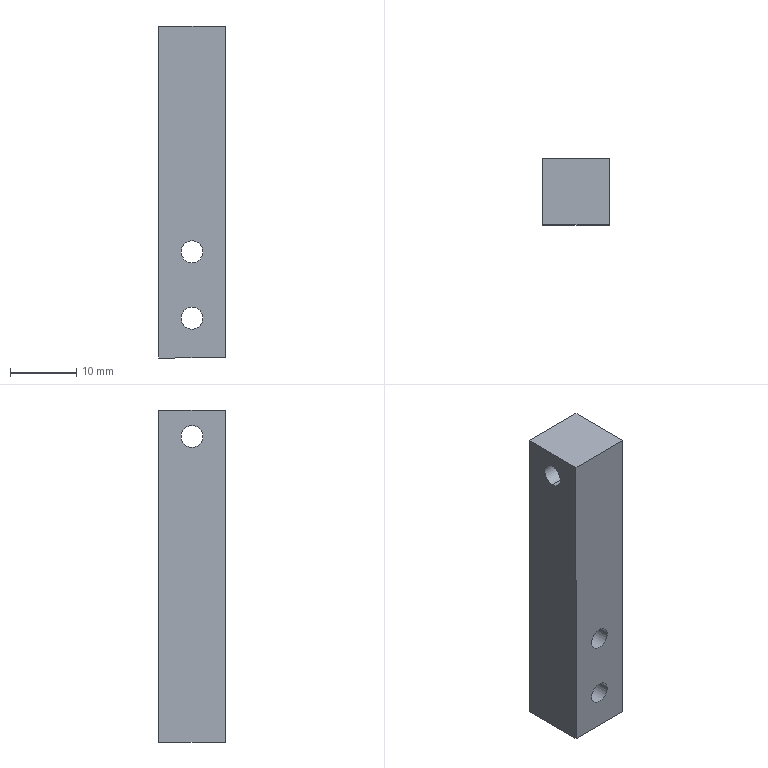Component | SolidWorks | CS021-A10-A024-1 | 1 solid | 12 faces | box 10 x 10 x 50 mm | volume 4743 mm3 | cylinder 6 | plane 6 | commonest cylinder face diameters 3.3 x6 | material AL6061
build123d program:
from build123d import *

# Parameters (mm, degrees)
SKETCH1_W                  = 50
SKETCH1_H                  = 10
BOSS_EXTRUDE1_DEPTH        = 5
F_3_3_3_3_DIAMETER_HOLE1_D = 3.3
M4_TAPPED_HOLE1_D          = 3.3


with BuildPart() as part:
    # Sketch1 → Boss-Extrude1 (new, symmetric)
    with BuildSketch(Plane.XY):
        Rectangle(SKETCH1_W, SKETCH1_H)
    extrude(amount=BOSS_EXTRUDE1_DEPTH, both=True)

    # 3.3 _3.3_ Diameter Hole1 (through all)
    with Locations(Plane(origin=(0, 5, 0), x_dir=(1, 0, 0), z_dir=(0, 1, 0))):
        with Locations((19, 0), (9, 0)):
            Hole(F_3_3_3_3_DIAMETER_HOLE1_D / 2)

    # M4 Tapped Hole1 (through all)
    with Locations(Plane.XY.offset(5)):
        with Locations((-21, 0)):
            Hole(M4_TAPPED_HOLE1_D / 2)


solid = part.part

# Placed as in the assembly
solid = solid.moved(Location((172.449, 93.817, -71), (0, 90, 0)))
STEP:
#1=CARTESIAN_POINT('',(6.592,3.694,-1.904));
#2=VERTEX_POINT('',#1);
#3=CARTESIAN_POINT('',(6.592,3.694,-2.033));
#4=VERTEX_POINT('',#3);
#5=CARTESIAN_POINT('',(6.592,3.694,-1.969));
#6=DIRECTION('',(1.,-0.,0.));
#7=DIRECTION('',(0.,0.,-1.));
#8=AXIS2_PLACEMENT_3D('',#5,#6,#7);
#9=CIRCLE('',#8,0.06496);
#10=EDGE_CURVE('',#2,#4,#9,.T.);
#11=ORIENTED_EDGE('',*,*,#10,.F.);
#12=CARTESIAN_POINT('',(6.986,3.694,-1.904));
#13=VERTEX_POINT('',#12);
#14=CARTESIAN_POINT('',(6.986,3.694,-1.904));
#15=DIRECTION('',(1.,-0.,0.));
#16=VECTOR('',#15,39.37);
#17=LINE('',#14,#16);
#18=EDGE_CURVE('',#2,#13,#17,.T.);
#19=ORIENTED_EDGE('',*,*,#18,.T.);
#20=CARTESIAN_POINT('',(6.986,3.694,-2.033));
#21=VERTEX_POINT('',#20);
#22=CARTESIAN_POINT('',(6.986,3.694,-1.969));
#23=DIRECTION('',(1.,-0.,0.));
#24=DIRECTION('',(0.,0.,-1.));
#25=AXIS2_PLACEMENT_3D('',#22,#23,#24);
#26=CIRCLE('',#25,0.06496);
#27=EDGE_CURVE('',#13,#21,#26,.T.);
#28=ORIENTED_EDGE('',*,*,#27,.T.);
#29=CARTESIAN_POINT('',(6.986,3.694,-2.033));
#30=DIRECTION('',(1.,-0.,0.));
#31=VECTOR('',#30,39.37);
#32=LINE('',#29,#31);
#33=EDGE_CURVE('',#4,#21,#32,.T.);
#34=ORIENTED_EDGE('',*,*,#33,.F.);
#35=EDGE_LOOP('',(#11,#19,#28,#34));
#36=FACE_OUTER_BOUND('',#35,.T.);
#37=CARTESIAN_POINT('',(6.986,3.694,-1.969));
#38=DIRECTION('',(1.,-0.,0.));
#39=DIRECTION('',(0.,0.,-1.));
#40=AXIS2_PLACEMENT_3D('',#37,#38,#39);
#41=CYLINDRICAL_SURFACE('',#40,0.06496);
#42=ADVANCED_FACE('',(#36),#41,.F.);
#43=CARTESIAN_POINT('',(6.724,3.497,-3.543));
#44=VERTEX_POINT('',#43);
#45=CARTESIAN_POINT('',(6.854,3.497,-3.543));
#46=VERTEX_POINT('',#45);
#47=CARTESIAN_POINT('',(6.789,3.497,-3.543));
#48=DIRECTION('',(0.,1.,-0.));
#49=DIRECTION('',(1.,0.,0.));
#50=AXIS2_PLACEMENT_3D('',#47,#48,#49);
#51=CIRCLE('',#50,0.06496);
#52=EDGE_CURVE('',#44,#46,#51,.T.);
#53=ORIENTED_EDGE('',*,*,#52,.F.);
#54=CARTESIAN_POINT('',(6.724,3.89,-3.543));
#55=VERTEX_POINT('',#54);
#56=CARTESIAN_POINT('',(6.724,3.89,-3.543));
#57=DIRECTION('',(0.,1.,-0.));
#58=VECTOR('',#57,39.37);
#59=LINE('',#56,#58);
#60=EDGE_CURVE('',#44,#55,#59,.T.);
#61=ORIENTED_EDGE('',*,*,#60,.T.);
#62=CARTESIAN_POINT('',(6.854,3.89,-3.543));
#63=VERTEX_POINT('',#62);
#64=CARTESIAN_POINT('',(6.789,3.89,-3.543));
#65=DIRECTION('',(0.,1.,-0.));
#66=DIRECTION('',(1.,0.,0.));
#67=AXIS2_PLACEMENT_3D('',#64,#65,#66);
#68=CIRCLE('',#67,0.06496);
#69=EDGE_CURVE('',#55,#63,#68,.T.);
#70=ORIENTED_EDGE('',*,*,#69,.T.);
#71=CARTESIAN_POINT('',(6.854,3.89,-3.543));
#72=DIRECTION('',(0.,1.,-0.));
#73=VECTOR('',#72,39.37);
#74=LINE('',#71,#73);
#75=EDGE_CURVE('',#46,#63,#74,.T.);
#76=ORIENTED_EDGE('',*,*,#75,.F.);
#77=EDGE_LOOP('',(#53,#61,#70,#76));
#78=FACE_OUTER_BOUND('',#77,.T.);
#79=CARTESIAN_POINT('',(6.789,3.89,-3.543));
#80=DIRECTION('',(0.,1.,-0.));
#81=DIRECTION('',(1.,0.,0.));
#82=AXIS2_PLACEMENT_3D('',#79,#80,#81);
#83=CYLINDRICAL_SURFACE('',#82,0.06496);
#84=ADVANCED_FACE('',(#78),#83,.F.);
#85=CARTESIAN_POINT('',(6.724,3.497,-3.15));
#86=VERTEX_POINT('',#85);
#87=CARTESIAN_POINT('',(6.854,3.497,-3.15));
#88=VERTEX_POINT('',#87);
#89=CARTESIAN_POINT('',(6.789,3.497,-3.15));
#90=DIRECTION('',(0.,1.,-0.));
#91=DIRECTION('',(1.,0.,0.));
#92=AXIS2_PLACEMENT_3D('',#89,#90,#91);
#93=CIRCLE('',#92,0.06496);
#94=EDGE_CURVE('',#86,#88,#93,.T.);
#95=ORIENTED_EDGE('',*,*,#94,.F.);
#96=CARTESIAN_POINT('',(6.724,3.89,-3.15));
#97=VERTEX_POINT('',#96);
#98=CARTESIAN_POINT('',(6.724,3.89,-3.15));
#99=DIRECTION('',(0.,1.,-0.));
#100=VECTOR('',#99,39.37);
#101=LINE('',#98,#100);
#102=EDGE_CURVE('',#86,#97,#101,.T.);
#103=ORIENTED_EDGE('',*,*,#102,.T.);
#104=CARTESIAN_POINT('',(6.854,3.89,-3.15));
#105=VERTEX_POINT('',#104);
#106=CARTESIAN_POINT('',(6.789,3.89,-3.15));
#107=DIRECTION('',(0.,1.,-0.));
#108=DIRECTION('',(1.,0.,0.));
#109=AXIS2_PLACEMENT_3D('',#106,#107,#108);
#110=CIRCLE('',#109,0.06496);
#111=EDGE_CURVE('',#97,#105,#110,.T.);
#112=ORIENTED_EDGE('',*,*,#111,.T.);
#113=CARTESIAN_POINT('',(6.854,3.89,-3.15));
#114=DIRECTION('',(0.,1.,-0.));
#115=VECTOR('',#114,39.37);
#116=LINE('',#113,#115);
#117=EDGE_CURVE('',#88,#105,#116,.T.);
#118=ORIENTED_EDGE('',*,*,#117,.F.);
#119=EDGE_LOOP('',(#95,#103,#112,#118));
#120=FACE_OUTER_BOUND('',#119,.T.);
#121=CARTESIAN_POINT('',(6.789,3.89,-3.15));
#122=DIRECTION('',(0.,1.,-0.));
#123=DIRECTION('',(1.,0.,0.));
#124=AXIS2_PLACEMENT_3D('',#121,#122,#123);
#125=CYLINDRICAL_SURFACE('',#124,0.06496);
#126=ADVANCED_FACE('',(#120),#125,.F.);
#127=CARTESIAN_POINT('',(6.592,3.497,-3.78));
#128=VERTEX_POINT('',#127);
#129=CARTESIAN_POINT('',(6.592,3.89,-3.78));
#130=VERTEX_POINT('',#129);
#131=CARTESIAN_POINT('',(6.592,3.497,-3.78));
#132=DIRECTION('',(0.,1.,-0.));
#133=VECTOR('',#132,39.37);
#134=LINE('',#131,#133);
#135=EDGE_CURVE('',#128,#130,#134,.T.);
#136=ORIENTED_EDGE('',*,*,#135,.T.);
#137=CARTESIAN_POINT('',(6.986,3.89,-3.78));
#138=VERTEX_POINT('',#137);
#139=CARTESIAN_POINT('',(6.986,3.89,-3.78));
#140=DIRECTION('',(-1.,0.,-0.));
#141=VECTOR('',#140,39.37);
#142=LINE('',#139,#141);
#143=EDGE_CURVE('',#138,#130,#142,.T.);
#144=ORIENTED_EDGE('',*,*,#143,.F.);
#145=CARTESIAN_POINT('',(6.986,3.497,-3.78));
#146=VERTEX_POINT('',#145);
#147=CARTESIAN_POINT('',(6.986,3.497,-3.78));
#148=DIRECTION('',(0.,1.,-0.));
#149=VECTOR('',#148,39.37);
#150=LINE('',#147,#149);
#151=EDGE_CURVE('',#146,#138,#150,.T.);
#152=ORIENTED_EDGE('',*,*,#151,.F.);
#153=CARTESIAN_POINT('',(6.986,3.497,-3.78));
#154=DIRECTION('',(-1.,0.,-0.));
#155=VECTOR('',#154,39.37);
#156=LINE('',#153,#155);
#157=EDGE_CURVE('',#146,#128,#156,.T.);
#158=ORIENTED_EDGE('',*,*,#157,.T.);
#159=EDGE_LOOP('',(#136,#144,#152,#158));
#160=FACE_OUTER_BOUND('',#159,.T.);
#161=CARTESIAN_POINT('',(6.986,3.497,-3.78));
#162=DIRECTION('',(-0.,0.,1.));
#163=DIRECTION('',(1.,-0.,0.));
#164=AXIS2_PLACEMENT_3D('',#161,#162,#163);
#165=PLANE('',#164);
#166=ADVANCED_FACE('',(#160),#165,.F.);
#167=CARTESIAN_POINT('',(6.789,3.89,-3.543));
#168=DIRECTION('',(0.,1.,-0.));
#169=DIRECTION('',(1.,0.,0.));
#170=AXIS2_PLACEMENT_3D('',#167,#168,#169);
#171=CIRCLE('',#170,0.06496);
#172=EDGE_CURVE('',#63,#55,#171,.T.);
#173=ORIENTED_EDGE('',*,*,#172,.F.);
#174=ORIENTED_EDGE('',*,*,#69,.F.);
#175=EDGE_LOOP('',(#173,#174));
#176=FACE_BOUND('',#175,.T.);
#177=CARTESIAN_POINT('',(6.789,3.89,-3.15));
#178=DIRECTION('',(0.,1.,-0.));
#179=DIRECTION('',(1.,0.,0.));
#180=AXIS2_PLACEMENT_3D('',#177,#178,#179);
#181=CIRCLE('',#180,0.06496);
#182=EDGE_CURVE('',#105,#97,#181,.T.);
#183=ORIENTED_EDGE('',*,*,#182,.F.);
#184=ORIENTED_EDGE('',*,*,#111,.F.);
#185=EDGE_LOOP('',(#183,#184));
#186=FACE_BOUND('',#185,.T.);
#187=CARTESIAN_POINT('',(6.592,3.89,-1.811));
#188=VERTEX_POINT('',#187);
#189=CARTESIAN_POINT('',(6.592,3.89,-1.811));
#190=DIRECTION('',(-0.,0.,1.));
#191=VECTOR('',#190,39.37);
#192=LINE('',#189,#191);
#193=EDGE_CURVE('',#130,#188,#192,.T.);
#194=ORIENTED_EDGE('',*,*,#193,.T.);
#195=CARTESIAN_POINT('',(6.986,3.89,-1.811));
#196=VERTEX_POINT('',#195);
#197=CARTESIAN_POINT('',(6.986,3.89,-1.811));
#198=DIRECTION('',(-1.,0.,-0.));
#199=VECTOR('',#198,39.37);
#200=LINE('',#197,#199);
#201=EDGE_CURVE('',#196,#188,#200,.T.);
#202=ORIENTED_EDGE('',*,*,#201,.F.);
#203=CARTESIAN_POINT('',(6.986,3.89,-1.811));
#204=DIRECTION('',(-0.,0.,1.));
#205=VECTOR('',#204,39.37);
#206=LINE('',#203,#205);
#207=EDGE_CURVE('',#138,#196,#206,.T.);
#208=ORIENTED_EDGE('',*,*,#207,.F.);
#209=ORIENTED_EDGE('',*,*,#143,.T.);
#210=EDGE_LOOP('',(#194,#202,#208,#209));
#211=FACE_OUTER_BOUND('',#210,.T.);
#212=CARTESIAN_POINT('',(6.986,3.89,-1.811));
#213=DIRECTION('',(-0.,-1.,0.));
#214=DIRECTION('',(-1.,0.,-0.));
#215=AXIS2_PLACEMENT_3D('',#212,#213,#214);
#216=PLANE('',#215);
#217=ADVANCED_FACE('',(#176,#186,#211),#216,.F.);
#218=CARTESIAN_POINT('',(6.592,3.497,-1.811));
#219=VERTEX_POINT('',#218);
#220=CARTESIAN_POINT('',(6.592,3.497,-1.811));
#221=DIRECTION('',(-0.,-1.,0.));
#222=VECTOR('',#221,39.37);
#223=LINE('',#220,#222);
#224=EDGE_CURVE('',#188,#219,#223,.T.);
#225=ORIENTED_EDGE('',*,*,#224,.T.);
#226=CARTESIAN_POINT('',(6.986,3.497,-1.811));
#227=VERTEX_POINT('',#226);
#228=CARTESIAN_POINT('',(6.986,3.497,-1.811));
#229=DIRECTION('',(-1.,0.,-0.));
#230=VECTOR('',#229,39.37);
#231=LINE('',#228,#230);
#232=EDGE_CURVE('',#227,#219,#231,.T.);
#233=ORIENTED_EDGE('',*,*,#232,.F.);
#234=CARTESIAN_POINT('',(6.986,3.497,-1.811));
#235=DIRECTION('',(-0.,-1.,0.));
#236=VECTOR('',#235,39.37);
#237=LINE('',#234,#236);
#238=EDGE_CURVE('',#196,#227,#237,.T.);
#239=ORIENTED_EDGE('',*,*,#238,.F.);
#240=ORIENTED_EDGE('',*,*,#201,.T.);
#241=EDGE_LOOP('',(#225,#233,#239,#240));
#242=FACE_OUTER_BOUND('',#241,.T.);
#243=CARTESIAN_POINT('',(6.986,3.497,-1.811));
#244=DIRECTION('',(0.,-0.,-1.));
#245=DIRECTION('',(-1.,0.,-0.));
#246=AXIS2_PLACEMENT_3D('',#243,#244,#245);
#247=PLANE('',#246);
#248=ADVANCED_FACE('',(#242),#247,.F.);
#249=CARTESIAN_POINT('',(6.789,3.497,-3.543));
#250=DIRECTION('',(0.,1.,-0.));
#251=DIRECTION('',(1.,0.,0.));
#252=AXIS2_PLACEMENT_3D('',#249,#250,#251);
#253=CIRCLE('',#252,0.06496);
#254=EDGE_CURVE('',#46,#44,#253,.T.);
#255=ORIENTED_EDGE('',*,*,#254,.T.);
#256=ORIENTED_EDGE('',*,*,#52,.T.);
#257=EDGE_LOOP('',(#255,#256));
#258=FACE_BOUND('',#257,.T.);
#259=CARTESIAN_POINT('',(6.789,3.497,-3.15));
#260=DIRECTION('',(0.,1.,-0.));
#261=DIRECTION('',(1.,0.,0.));
#262=AXIS2_PLACEMENT_3D('',#259,#260,#261);
#263=CIRCLE('',#262,0.06496);
#264=EDGE_CURVE('',#88,#86,#263,.T.);
#265=ORIENTED_EDGE('',*,*,#264,.T.);
#266=ORIENTED_EDGE('',*,*,#94,.T.);
#267=EDGE_LOOP('',(#265,#266));
#268=FACE_BOUND('',#267,.T.);
#269=CARTESIAN_POINT('',(6.592,3.497,-1.811));
#270=DIRECTION('',(0.,-0.,-1.));
#271=VECTOR('',#270,39.37);
#272=LINE('',#269,#271);
#273=EDGE_CURVE('',#219,#128,#272,.T.);
#274=ORIENTED_EDGE('',*,*,#273,.T.);
#275=ORIENTED_EDGE('',*,*,#157,.F.);
#276=CARTESIAN_POINT('',(6.986,3.497,-1.811));
#277=DIRECTION('',(0.,-0.,-1.));
#278=VECTOR('',#277,39.37);
#279=LINE('',#276,#278);
#280=EDGE_CURVE('',#227,#146,#279,.T.);
#281=ORIENTED_EDGE('',*,*,#280,.F.);
#282=ORIENTED_EDGE('',*,*,#232,.T.);
#283=EDGE_LOOP('',(#274,#275,#281,#282));
#284=FACE_OUTER_BOUND('',#283,.T.);
#285=CARTESIAN_POINT('',(6.986,3.497,-1.811));
#286=DIRECTION('',(0.,1.,-0.));
#287=DIRECTION('',(1.,-0.,0.));
#288=AXIS2_PLACEMENT_3D('',#285,#286,#287);
#289=PLANE('',#288);
#290=ADVANCED_FACE('',(#258,#268,#284),#289,.F.);
#291=CARTESIAN_POINT('',(6.986,3.694,-1.969));
#292=DIRECTION('',(1.,-0.,0.));
#293=DIRECTION('',(0.,0.,-1.));
#294=AXIS2_PLACEMENT_3D('',#291,#292,#293);
#295=CIRCLE('',#294,0.06496);
#296=EDGE_CURVE('',#21,#13,#295,.T.);
#297=ORIENTED_EDGE('',*,*,#296,.F.);
#298=ORIENTED_EDGE('',*,*,#27,.F.);
#299=EDGE_LOOP('',(#297,#298));
#300=FACE_BOUND('',#299,.T.);
#301=ORIENTED_EDGE('',*,*,#151,.T.);
#302=ORIENTED_EDGE('',*,*,#207,.T.);
#303=ORIENTED_EDGE('',*,*,#238,.T.);
#304=ORIENTED_EDGE('',*,*,#280,.T.);
#305=EDGE_LOOP('',(#301,#302,#303,#304));
#306=FACE_OUTER_BOUND('',#305,.T.);
#307=CARTESIAN_POINT('',(6.986,3.694,-2.795));
#308=DIRECTION('',(-1.,0.,-0.));
#309=DIRECTION('',(-0.,0.,1.));
#310=AXIS2_PLACEMENT_3D('',#307,#308,#309);
#311=PLANE('',#310);
#312=ADVANCED_FACE('',(#300,#306),#311,.F.);
#313=CARTESIAN_POINT('',(6.592,3.694,-1.969));
#314=DIRECTION('',(1.,-0.,0.));
#315=DIRECTION('',(0.,0.,-1.));
#316=AXIS2_PLACEMENT_3D('',#313,#314,#315);
#317=CIRCLE('',#316,0.06496);
#318=EDGE_CURVE('',#4,#2,#317,.T.);
#319=ORIENTED_EDGE('',*,*,#318,.T.);
#320=ORIENTED_EDGE('',*,*,#10,.T.);
#321=EDGE_LOOP('',(#319,#320));
#322=FACE_BOUND('',#321,.T.);
#323=ORIENTED_EDGE('',*,*,#135,.F.);
#324=ORIENTED_EDGE('',*,*,#273,.F.);
#325=ORIENTED_EDGE('',*,*,#224,.F.);
#326=ORIENTED_EDGE('',*,*,#193,.F.);
#327=EDGE_LOOP('',(#323,#324,#325,#326));
#328=FACE_OUTER_BOUND('',#327,.T.);
#329=CARTESIAN_POINT('',(6.592,3.694,-2.795));
#330=DIRECTION('',(-1.,0.,-0.));
#331=DIRECTION('',(-0.,0.,1.));
#332=AXIS2_PLACEMENT_3D('',#329,#330,#331);
#333=PLANE('',#332);
#334=ADVANCED_FACE('',(#322,#328),#333,.T.);
#335=ORIENTED_EDGE('',*,*,#102,.F.);
#336=ORIENTED_EDGE('',*,*,#264,.F.);
#337=ORIENTED_EDGE('',*,*,#117,.T.);
#338=ORIENTED_EDGE('',*,*,#182,.T.);
#339=EDGE_LOOP('',(#335,#336,#337,#338));
#340=FACE_OUTER_BOUND('',#339,.T.);
#341=CARTESIAN_POINT('',(6.789,3.89,-3.15));
#342=DIRECTION('',(0.,1.,-0.));
#343=DIRECTION('',(1.,0.,0.));
#344=AXIS2_PLACEMENT_3D('',#341,#342,#343);
#345=CYLINDRICAL_SURFACE('',#344,0.06496);
#346=ADVANCED_FACE('',(#340),#345,.F.);
#347=ORIENTED_EDGE('',*,*,#60,.F.);
#348=ORIENTED_EDGE('',*,*,#254,.F.);
#349=ORIENTED_EDGE('',*,*,#75,.T.);
#350=ORIENTED_EDGE('',*,*,#172,.T.);
#351=EDGE_LOOP('',(#347,#348,#349,#350));
#352=FACE_OUTER_BOUND('',#351,.T.);
#353=CARTESIAN_POINT('',(6.789,3.89,-3.543));
#354=DIRECTION('',(0.,1.,-0.));
#355=DIRECTION('',(1.,0.,0.));
#356=AXIS2_PLACEMENT_3D('',#353,#354,#355);
#357=CYLINDRICAL_SURFACE('',#356,0.06496);
#358=ADVANCED_FACE('',(#352),#357,.F.);
#359=ORIENTED_EDGE('',*,*,#18,.F.);
#360=ORIENTED_EDGE('',*,*,#318,.F.);
#361=ORIENTED_EDGE('',*,*,#33,.T.);
#362=ORIENTED_EDGE('',*,*,#296,.T.);
#363=EDGE_LOOP('',(#359,#360,#361,#362));
#364=FACE_OUTER_BOUND('',#363,.T.);
#365=CARTESIAN_POINT('',(6.986,3.694,-1.969));
#366=DIRECTION('',(1.,-0.,0.));
#367=DIRECTION('',(0.,0.,-1.));
#368=AXIS2_PLACEMENT_3D('',#365,#366,#367);
#369=CYLINDRICAL_SURFACE('',#368,0.06496);
#370=ADVANCED_FACE('',(#364),#369,.F.);
#371=CLOSED_SHELL('',(#42,#84,#126,#166,#217,#248,#290,#312,#334,#346,#358,#370));
#372=MANIFOLD_SOLID_BREP('',#371);
#373=CARTESIAN_POINT('',(0.,0.,0.));
#374=DIRECTION('',(0.,0.,1.));
#375=DIRECTION('',(1.,0.,0.));
#376=AXIS2_PLACEMENT_3D('',#373,#374,#375);
#377=(LENGTH_UNIT()NAMED_UNIT(*)SI_UNIT($,.METRE.));
#378=LENGTH_MEASURE_WITH_UNIT(LENGTH_MEASURE(0.0254),#377);
#379=DIMENSIONAL_EXPONENTS(1.,0.,0.,0.,0.,0.,0.);
#380=(CONVERSION_BASED_UNIT('',#378)LENGTH_UNIT()NAMED_UNIT(#379));
#381=UNCERTAINTY_MEASURE_WITH_UNIT(LENGTH_MEASURE(0.00001),#380,'','');
#382=(NAMED_UNIT(*)PLANE_ANGLE_UNIT()SI_UNIT($,.RADIAN.));
#383=(NAMED_UNIT(*)SI_UNIT($,.STERADIAN.)SOLID_ANGLE_UNIT());
#384=(GEOMETRIC_REPRESENTATION_CONTEXT(3)GLOBAL_UNCERTAINTY_ASSIGNED_CONTEXT((#381))GLOBAL_UNIT_ASSIGNED_CONTEXT((#380,#382,#383))REPRESENTATION_CONTEXT('',''));
#385=ADVANCED_BREP_SHAPE_REPRESENTATION('',(#372,#376),#384);
#386=COLOUR_RGB('',0.7922,0.8196,0.9333);
#387=FILL_AREA_STYLE_COLOUR('',#386);
#388=FILL_AREA_STYLE('',(#387));
#389=SURFACE_STYLE_FILL_AREA(#388);
#390=SURFACE_SIDE_STYLE('',(#389));
#391=SURFACE_STYLE_USAGE(.BOTH.,#390);
#392=PRESENTATION_STYLE_ASSIGNMENT((#391));
#393=STYLED_ITEM('',(#392),#372);
#394=(LENGTH_UNIT()NAMED_UNIT(*)SI_UNIT($,.METRE.));
#395=LENGTH_MEASURE_WITH_UNIT(LENGTH_MEASURE(0.0254),#394);
#396=DIMENSIONAL_EXPONENTS(1.,0.,0.,0.,0.,0.,0.);
#397=(CONVERSION_BASED_UNIT('',#395)LENGTH_UNIT()NAMED_UNIT(#396));
#398=UNCERTAINTY_MEASURE_WITH_UNIT(LENGTH_MEASURE(0.00001),#397,'','');
#399=(NAMED_UNIT(*)PLANE_ANGLE_UNIT()SI_UNIT($,.RADIAN.));
#400=(NAMED_UNIT(*)SI_UNIT($,.STERADIAN.)SOLID_ANGLE_UNIT());
#401=(GEOMETRIC_REPRESENTATION_CONTEXT(3)GLOBAL_UNCERTAINTY_ASSIGNED_CONTEXT((#398))GLOBAL_UNIT_ASSIGNED_CONTEXT((#397,#399,#400))REPRESENTATION_CONTEXT('',''));
#402=MECHANICAL_DESIGN_GEOMETRIC_PRESENTATION_REPRESENTATION('',(#393),#401);
#403=PRESENTATION_LAYER_ASSIGNMENT('','',(#393));